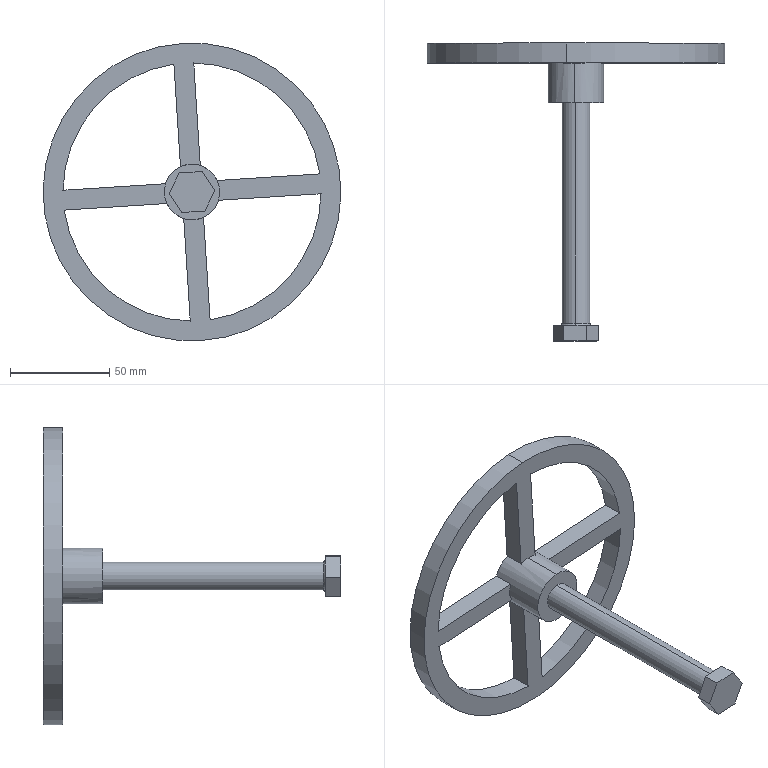Component | SolidWorks | adjuster roll-1 | 1 solid | 31 faces | box 150 x 150 x 150 mm | volume 102973 mm3 | plane 19 | cylinder 10 | torus 2 | commonest cylinder face diameters 130 x4 150 x2 28 x2 14 x2
STEP:
#1=COLOUR_RGB('',0.7922,0.8196,0.9333);
#2=FILL_AREA_STYLE_COLOUR('',#1);
#3=FILL_AREA_STYLE('',(#2));
#4=SURFACE_STYLE_FILL_AREA(#3);
#5=SURFACE_SIDE_STYLE('',(#4));
#6=SURFACE_STYLE_USAGE(.BOTH.,#5);
#7=PRESENTATION_STYLE_ASSIGNMENT((#6));
#8=CARTESIAN_POINT('',(-0.01998,5.433,1.102));
#9=VERTEX_POINT('',#8);
#10=CARTESIAN_POINT('',(0.01998,5.433,0.4731));
#11=VERTEX_POINT('',#10);
#12=CARTESIAN_POINT('',(0.,5.433,0.7874));
#13=DIRECTION('',(0.,-1.,0.));
#14=DIRECTION('',(0.06342,0.,-0.998));
#15=AXIS2_PLACEMENT_3D('',#12,#13,#14);
#16=CIRCLE('',#15,0.315);
#17=EDGE_CURVE('',#9,#11,#16,.T.);
#18=ORIENTED_EDGE('',*,*,#17,.F.);
#19=CARTESIAN_POINT('',(-0.01748,5.472,1.062));
#20=VERTEX_POINT('',#19);
#21=CARTESIAN_POINT('',(-0.01998,5.472,1.102));
#22=DIRECTION('',(0.998,0.,0.06342));
#23=DIRECTION('',(0.06342,0.,-0.998));
#24=AXIS2_PLACEMENT_3D('',#21,#22,#23);
#25=CIRCLE('',#24,0.03937);
#26=EDGE_CURVE('',#9,#20,#25,.T.);
#27=ORIENTED_EDGE('',*,*,#26,.T.);
#28=CARTESIAN_POINT('',(0.01748,5.472,0.5124));
#29=VERTEX_POINT('',#28);
#30=CARTESIAN_POINT('',(0.,5.472,0.7874));
#31=DIRECTION('',(0.,1.,0.));
#32=DIRECTION('',(0.06342,0.,-0.998));
#33=AXIS2_PLACEMENT_3D('',#30,#31,#32);
#34=CIRCLE('',#33,0.2756);
#35=EDGE_CURVE('',#29,#20,#34,.T.);
#36=ORIENTED_EDGE('',*,*,#35,.F.);
#37=CARTESIAN_POINT('',(0.01998,5.472,0.4731));
#38=DIRECTION('',(-0.998,0.,-0.06342));
#39=DIRECTION('',(-0.06342,0.,0.998));
#40=AXIS2_PLACEMENT_3D('',#37,#38,#39);
#41=CIRCLE('',#40,0.03937);
#42=EDGE_CURVE('',#11,#29,#41,.T.);
#43=ORIENTED_EDGE('',*,*,#42,.F.);
#44=EDGE_LOOP('',(#18,#27,#36,#43));
#45=FACE_OUTER_BOUND('',#44,.T.);
#46=CARTESIAN_POINT('',(0.,5.472,0.7874));
#47=DIRECTION('',(0.,-1.,0.));
#48=DIRECTION('',(0.06342,0.,-0.998));
#49=AXIS2_PLACEMENT_3D('',#46,#47,#48);
#50=TOROIDAL_SURFACE('',#49,0.315,0.03937);
#51=ADVANCED_FACE('',(#45),#50,.F.);
#52=CARTESIAN_POINT('',(-0.1873,11.024,3.734));
#53=VERTEX_POINT('',#52);
#54=CARTESIAN_POINT('',(0.1873,11.024,-2.159));
#55=VERTEX_POINT('',#54);
#56=CARTESIAN_POINT('',(0.,11.024,0.7874));
#57=DIRECTION('',(0.,1.,0.));
#58=DIRECTION('',(-0.06342,0.,0.998));
#59=AXIS2_PLACEMENT_3D('',#56,#57,#58);
#60=CIRCLE('',#59,2.953);
#61=EDGE_CURVE('',#53,#55,#60,.T.);
#62=ORIENTED_EDGE('',*,*,#61,.F.);
#63=CARTESIAN_POINT('',(-0.1873,10.63,3.734));
#64=VERTEX_POINT('',#63);
#65=CARTESIAN_POINT('',(-0.1873,11.024,3.734));
#66=DIRECTION('',(0.,-1.,0.));
#67=VECTOR('',#66,39.37);
#68=LINE('',#65,#67);
#69=EDGE_CURVE('',#53,#64,#68,.T.);
#70=ORIENTED_EDGE('',*,*,#69,.T.);
#71=CARTESIAN_POINT('',(0.1873,10.63,-2.159));
#72=VERTEX_POINT('',#71);
#73=CARTESIAN_POINT('',(0.,10.63,0.7874));
#74=DIRECTION('',(0.,1.,0.));
#75=DIRECTION('',(-0.06342,0.,0.998));
#76=AXIS2_PLACEMENT_3D('',#73,#74,#75);
#77=CIRCLE('',#76,2.953);
#78=EDGE_CURVE('',#64,#72,#77,.T.);
#79=ORIENTED_EDGE('',*,*,#78,.T.);
#80=CARTESIAN_POINT('',(0.1873,11.024,-2.159));
#81=DIRECTION('',(0.,-1.,0.));
#82=VECTOR('',#81,39.37);
#83=LINE('',#80,#82);
#84=EDGE_CURVE('',#55,#72,#83,.T.);
#85=ORIENTED_EDGE('',*,*,#84,.F.);
#86=EDGE_LOOP('',(#62,#70,#79,#85));
#87=FACE_OUTER_BOUND('',#86,.T.);
#88=CARTESIAN_POINT('',(0.,11.024,0.7874));
#89=DIRECTION('',(0.,-1.,0.));
#90=DIRECTION('',(0.06342,0.,-0.998));
#91=AXIS2_PLACEMENT_3D('',#88,#89,#90);
#92=CYLINDRICAL_SURFACE('',#91,2.953);
#93=ADVANCED_FACE('',(#87),#92,.T.);
#94=CARTESIAN_POINT('',(-0.03496,10.63,1.337));
#95=VERTEX_POINT('',#94);
#96=CARTESIAN_POINT('',(0.1638,10.63,1.314));
#97=VERTEX_POINT('',#96);
#98=CARTESIAN_POINT('',(0.,10.63,0.7874));
#99=DIRECTION('',(0.,1.,0.));
#100=DIRECTION('',(-0.06342,0.,0.998));
#101=AXIS2_PLACEMENT_3D('',#98,#99,#100);
#102=CIRCLE('',#101,0.5512);
#103=EDGE_CURVE('',#95,#97,#102,.T.);
#104=ORIENTED_EDGE('',*,*,#103,.F.);
#105=CARTESIAN_POINT('',(-0.03496,9.843,1.337));
#106=VERTEX_POINT('',#105);
#107=CARTESIAN_POINT('',(-0.03496,10.63,1.337));
#108=DIRECTION('',(0.,-1.,0.));
#109=VECTOR('',#108,39.37);
#110=LINE('',#107,#109);
#111=EDGE_CURVE('',#95,#106,#110,.T.);
#112=ORIENTED_EDGE('',*,*,#111,.T.);
#113=CARTESIAN_POINT('',(0.03496,9.843,0.2373));
#114=VERTEX_POINT('',#113);
#115=CARTESIAN_POINT('',(0.,9.843,0.7874));
#116=DIRECTION('',(0.,1.,0.));
#117=DIRECTION('',(-0.06342,0.,0.998));
#118=AXIS2_PLACEMENT_3D('',#115,#116,#117);
#119=CIRCLE('',#118,0.5512);
#120=EDGE_CURVE('',#106,#114,#119,.T.);
#121=ORIENTED_EDGE('',*,*,#120,.T.);
#122=CARTESIAN_POINT('',(0.03496,10.63,0.2373));
#123=VERTEX_POINT('',#122);
#124=CARTESIAN_POINT('',(0.03496,10.63,0.2373));
#125=DIRECTION('',(0.,-1.,0.));
#126=VECTOR('',#125,39.37);
#127=LINE('',#124,#126);
#128=EDGE_CURVE('',#123,#114,#127,.T.);
#129=ORIENTED_EDGE('',*,*,#128,.F.);
#130=CARTESIAN_POINT('',(0.2291,10.63,0.2861));
#131=VERTEX_POINT('',#130);
#132=CARTESIAN_POINT('',(0.,10.63,0.7874));
#133=DIRECTION('',(0.,1.,0.));
#134=DIRECTION('',(-0.06342,0.,0.998));
#135=AXIS2_PLACEMENT_3D('',#132,#133,#134);
#136=CIRCLE('',#135,0.5512);
#137=EDGE_CURVE('',#131,#123,#136,.T.);
#138=ORIENTED_EDGE('',*,*,#137,.F.);
#139=CARTESIAN_POINT('',(0.2291,11.024,0.2861));
#140=VERTEX_POINT('',#139);
#141=CARTESIAN_POINT('',(0.2291,11.024,0.2861));
#142=DIRECTION('',(0.,-1.,0.));
#143=VECTOR('',#142,39.37);
#144=LINE('',#141,#143);
#145=EDGE_CURVE('',#140,#131,#144,.T.);
#146=ORIENTED_EDGE('',*,*,#145,.F.);
#147=CARTESIAN_POINT('',(0.5263,11.024,0.6236));
#148=VERTEX_POINT('',#147);
#149=CARTESIAN_POINT('',(0.,11.024,0.7874));
#150=DIRECTION('',(0.,1.,0.));
#151=DIRECTION('',(-0.06342,0.,0.998));
#152=AXIS2_PLACEMENT_3D('',#149,#150,#151);
#153=CIRCLE('',#152,0.5512);
#154=EDGE_CURVE('',#148,#140,#153,.T.);
#155=ORIENTED_EDGE('',*,*,#154,.F.);
#156=CARTESIAN_POINT('',(0.5263,10.63,0.6236));
#157=VERTEX_POINT('',#156);
#158=CARTESIAN_POINT('',(0.5263,11.024,0.6236));
#159=DIRECTION('',(0.,-1.,0.));
#160=VECTOR('',#159,39.37);
#161=LINE('',#158,#160);
#162=EDGE_CURVE('',#148,#157,#161,.T.);
#163=ORIENTED_EDGE('',*,*,#162,.T.);
#164=CARTESIAN_POINT('',(0.5013,10.63,1.017));
#165=VERTEX_POINT('',#164);
#166=CARTESIAN_POINT('',(0.,10.63,0.7874));
#167=DIRECTION('',(0.,1.,0.));
#168=DIRECTION('',(-0.06342,0.,0.998));
#169=AXIS2_PLACEMENT_3D('',#166,#167,#168);
#170=CIRCLE('',#169,0.5512);
#171=EDGE_CURVE('',#165,#157,#170,.T.);
#172=ORIENTED_EDGE('',*,*,#171,.F.);
#173=CARTESIAN_POINT('',(0.5013,11.024,1.017));
#174=VERTEX_POINT('',#173);
#175=CARTESIAN_POINT('',(0.5013,11.024,1.017));
#176=DIRECTION('',(0.,-1.,0.));
#177=VECTOR('',#176,39.37);
#178=LINE('',#175,#177);
#179=EDGE_CURVE('',#174,#165,#178,.T.);
#180=ORIENTED_EDGE('',*,*,#179,.F.);
#181=CARTESIAN_POINT('',(0.1638,11.024,1.314));
#182=VERTEX_POINT('',#181);
#183=CARTESIAN_POINT('',(0.,11.024,0.7874));
#184=DIRECTION('',(0.,1.,0.));
#185=DIRECTION('',(-0.06342,0.,0.998));
#186=AXIS2_PLACEMENT_3D('',#183,#184,#185);
#187=CIRCLE('',#186,0.5512);
#188=EDGE_CURVE('',#182,#174,#187,.T.);
#189=ORIENTED_EDGE('',*,*,#188,.F.);
#190=CARTESIAN_POINT('',(0.1638,11.024,1.314));
#191=DIRECTION('',(0.,-1.,0.));
#192=VECTOR('',#191,39.37);
#193=LINE('',#190,#192);
#194=EDGE_CURVE('',#182,#97,#193,.T.);
#195=ORIENTED_EDGE('',*,*,#194,.T.);
#196=EDGE_LOOP('',(#104,#112,#121,#129,#138,#146,#155,#163,#172,#180,#189,#195));
#197=FACE_OUTER_BOUND('',#196,.T.);
#198=CARTESIAN_POINT('',(0.,10.63,0.7874));
#199=DIRECTION('',(0.,-1.,0.));
#200=DIRECTION('',(0.06342,0.,-0.998));
#201=AXIS2_PLACEMENT_3D('',#198,#199,#200);
#202=CYLINDRICAL_SURFACE('',#201,0.5512);
#203=ADVANCED_FACE('',(#197),#202,.T.);
#204=CARTESIAN_POINT('',(-0.01748,9.843,1.062));
#205=VERTEX_POINT('',#204);
#206=CARTESIAN_POINT('',(0.01748,9.843,0.5124));
#207=VERTEX_POINT('',#206);
#208=CARTESIAN_POINT('',(0.,9.843,0.7874));
#209=DIRECTION('',(0.,1.,0.));
#210=DIRECTION('',(-0.06342,0.,0.998));
#211=AXIS2_PLACEMENT_3D('',#208,#209,#210);
#212=CIRCLE('',#211,0.2756);
#213=EDGE_CURVE('',#205,#207,#212,.T.);
#214=ORIENTED_EDGE('',*,*,#213,.F.);
#215=CARTESIAN_POINT('',(-0.01748,9.843,1.062));
#216=DIRECTION('',(0.,-1.,0.));
#217=VECTOR('',#216,39.37);
#218=LINE('',#215,#217);
#219=EDGE_CURVE('',#205,#20,#218,.T.);
#220=ORIENTED_EDGE('',*,*,#219,.T.);
#221=CARTESIAN_POINT('',(0.,5.472,0.7874));
#222=DIRECTION('',(0.,1.,0.));
#223=DIRECTION('',(0.06342,0.,-0.998));
#224=AXIS2_PLACEMENT_3D('',#221,#222,#223);
#225=CIRCLE('',#224,0.2756);
#226=EDGE_CURVE('',#20,#29,#225,.T.);
#227=ORIENTED_EDGE('',*,*,#226,.T.);
#228=CARTESIAN_POINT('',(0.01748,9.843,0.5124));
#229=DIRECTION('',(0.,-1.,0.));
#230=VECTOR('',#229,39.37);
#231=LINE('',#228,#230);
#232=EDGE_CURVE('',#207,#29,#231,.T.);
#233=ORIENTED_EDGE('',*,*,#232,.F.);
#234=EDGE_LOOP('',(#214,#220,#227,#233));
#235=FACE_OUTER_BOUND('',#234,.T.);
#236=CARTESIAN_POINT('',(0.,9.843,0.7874));
#237=DIRECTION('',(0.,-1.,0.));
#238=DIRECTION('',(0.06342,0.,-0.998));
#239=AXIS2_PLACEMENT_3D('',#236,#237,#238);
#240=CYLINDRICAL_SURFACE('',#239,0.2756);
#241=ADVANCED_FACE('',(#235),#240,.T.);
#242=CARTESIAN_POINT('',(-0.1638,11.024,0.2611));
#243=VERTEX_POINT('',#242);
#244=CARTESIAN_POINT('',(-0.1638,10.63,0.2611));
#245=VERTEX_POINT('',#244);
#246=CARTESIAN_POINT('',(-0.1638,11.024,0.2611));
#247=DIRECTION('',(0.,-1.,0.));
#248=VECTOR('',#247,39.37);
#249=LINE('',#246,#248);
#250=EDGE_CURVE('',#243,#245,#249,.T.);
#251=ORIENTED_EDGE('',*,*,#250,.F.);
#252=CARTESIAN_POINT('',(-0.03463,11.024,-1.771));
#253=VERTEX_POINT('',#252);
#254=CARTESIAN_POINT('',(-0.1965,11.024,0.7749));
#255=DIRECTION('',(0.06342,0.,-0.998));
#256=VECTOR('',#255,39.37);
#257=LINE('',#254,#256);
#258=EDGE_CURVE('',#243,#253,#257,.T.);
#259=ORIENTED_EDGE('',*,*,#258,.T.);
#260=CARTESIAN_POINT('',(-0.03463,10.63,-1.771));
#261=VERTEX_POINT('',#260);
#262=CARTESIAN_POINT('',(-0.03463,7.3,-1.771));
#263=DIRECTION('',(0.,1.,0.));
#264=VECTOR('',#263,39.37);
#265=LINE('',#262,#264);
#266=EDGE_CURVE('',#261,#253,#265,.T.);
#267=ORIENTED_EDGE('',*,*,#266,.F.);
#268=CARTESIAN_POINT('',(-0.1965,10.63,0.7749));
#269=DIRECTION('',(-0.06342,0.,0.998));
#270=VECTOR('',#269,39.37);
#271=LINE('',#268,#270);
#272=EDGE_CURVE('',#261,#245,#271,.T.);
#273=ORIENTED_EDGE('',*,*,#272,.T.);
#274=EDGE_LOOP('',(#251,#259,#267,#273));
#275=FACE_OUTER_BOUND('',#274,.T.);
#276=CARTESIAN_POINT('',(-0.1965,7.3,0.7749));
#277=DIRECTION('',(0.998,0.,0.06342));
#278=DIRECTION('',(0.06342,0.,-0.998));
#279=AXIS2_PLACEMENT_3D('',#276,#277,#278);
#280=PLANE('',#279);
#281=ADVANCED_FACE('',(#275),#280,.F.);
#282=CARTESIAN_POINT('',(-0.5013,11.024,0.5583));
#283=VERTEX_POINT('',#282);
#284=CARTESIAN_POINT('',(-2.534,11.024,0.4291));
#285=VERTEX_POINT('',#284);
#286=CARTESIAN_POINT('',(0.01248,11.024,0.5909));
#287=DIRECTION('',(-0.998,0.,-0.06342));
#288=VECTOR('',#287,39.37);
#289=LINE('',#286,#288);
#290=EDGE_CURVE('',#283,#285,#289,.T.);
#291=ORIENTED_EDGE('',*,*,#290,.F.);
#292=CARTESIAN_POINT('',(-0.5013,10.63,0.5583));
#293=VERTEX_POINT('',#292);
#294=CARTESIAN_POINT('',(-0.5013,11.024,0.5583));
#295=DIRECTION('',(0.,-1.,0.));
#296=VECTOR('',#295,39.37);
#297=LINE('',#294,#296);
#298=EDGE_CURVE('',#283,#293,#297,.T.);
#299=ORIENTED_EDGE('',*,*,#298,.T.);
#300=CARTESIAN_POINT('',(-2.534,10.63,0.4291));
#301=VERTEX_POINT('',#300);
#302=CARTESIAN_POINT('',(0.01248,10.63,0.5909));
#303=DIRECTION('',(0.998,0.,0.06342));
#304=VECTOR('',#303,39.37);
#305=LINE('',#302,#304);
#306=EDGE_CURVE('',#301,#293,#305,.T.);
#307=ORIENTED_EDGE('',*,*,#306,.F.);
#308=CARTESIAN_POINT('',(-2.534,7.3,0.4291));
#309=DIRECTION('',(0.,1.,0.));
#310=VECTOR('',#309,39.37);
#311=LINE('',#308,#310);
#312=EDGE_CURVE('',#301,#285,#311,.T.);
#313=ORIENTED_EDGE('',*,*,#312,.T.);
#314=EDGE_LOOP('',(#291,#299,#307,#313));
#315=FACE_OUTER_BOUND('',#314,.T.);
#316=CARTESIAN_POINT('',(0.01248,7.3,0.5909));
#317=DIRECTION('',(0.06342,0.,-0.998));
#318=DIRECTION('',(-0.998,0.,-0.06342));
#319=AXIS2_PLACEMENT_3D('',#316,#317,#318);
#320=PLANE('',#319);
#321=ADVANCED_FACE('',(#315),#320,.T.);
#322=CARTESIAN_POINT('',(-0.5263,11.024,0.9512));
#323=VERTEX_POINT('',#322);
#324=CARTESIAN_POINT('',(-0.5263,10.63,0.9512));
#325=VERTEX_POINT('',#324);
#326=CARTESIAN_POINT('',(-0.5263,11.024,0.9512));
#327=DIRECTION('',(0.,-1.,0.));
#328=VECTOR('',#327,39.37);
#329=LINE('',#326,#328);
#330=EDGE_CURVE('',#323,#325,#329,.T.);
#331=ORIENTED_EDGE('',*,*,#330,.F.);
#332=CARTESIAN_POINT('',(-2.559,11.024,0.822));
#333=VERTEX_POINT('',#332);
#334=CARTESIAN_POINT('',(-0.01248,11.024,0.9839));
#335=DIRECTION('',(-0.998,0.,-0.06342));
#336=VECTOR('',#335,39.37);
#337=LINE('',#334,#336);
#338=EDGE_CURVE('',#323,#333,#337,.T.);
#339=ORIENTED_EDGE('',*,*,#338,.T.);
#340=CARTESIAN_POINT('',(-2.559,10.63,0.822));
#341=VERTEX_POINT('',#340);
#342=CARTESIAN_POINT('',(-2.559,7.3,0.822));
#343=DIRECTION('',(0.,1.,0.));
#344=VECTOR('',#343,39.37);
#345=LINE('',#342,#344);
#346=EDGE_CURVE('',#341,#333,#345,.T.);
#347=ORIENTED_EDGE('',*,*,#346,.F.);
#348=CARTESIAN_POINT('',(-0.01248,10.63,0.9839));
#349=DIRECTION('',(0.998,0.,0.06342));
#350=VECTOR('',#349,39.37);
#351=LINE('',#348,#350);
#352=EDGE_CURVE('',#341,#325,#351,.T.);
#353=ORIENTED_EDGE('',*,*,#352,.T.);
#354=EDGE_LOOP('',(#331,#339,#347,#353));
#355=FACE_OUTER_BOUND('',#354,.T.);
#356=CARTESIAN_POINT('',(-0.01248,7.3,0.9839));
#357=DIRECTION('',(0.06342,0.,-0.998));
#358=DIRECTION('',(-0.998,0.,-0.06342));
#359=AXIS2_PLACEMENT_3D('',#356,#357,#358);
#360=PLANE('',#359);
#361=ADVANCED_FACE('',(#355),#360,.F.);
#362=CARTESIAN_POINT('',(-0.2291,11.024,1.289));
#363=VERTEX_POINT('',#362);
#364=CARTESIAN_POINT('',(-0.3583,11.024,3.321));
#365=VERTEX_POINT('',#364);
#366=CARTESIAN_POINT('',(-0.1965,11.024,0.7749));
#367=DIRECTION('',(-0.06342,0.,0.998));
#368=VECTOR('',#367,39.37);
#369=LINE('',#366,#368);
#370=EDGE_CURVE('',#363,#365,#369,.T.);
#371=ORIENTED_EDGE('',*,*,#370,.F.);
#372=CARTESIAN_POINT('',(-0.2291,10.63,1.289));
#373=VERTEX_POINT('',#372);
#374=CARTESIAN_POINT('',(-0.2291,11.024,1.289));
#375=DIRECTION('',(0.,-1.,0.));
#376=VECTOR('',#375,39.37);
#377=LINE('',#374,#376);
#378=EDGE_CURVE('',#363,#373,#377,.T.);
#379=ORIENTED_EDGE('',*,*,#378,.T.);
#380=CARTESIAN_POINT('',(-0.3583,10.63,3.321));
#381=VERTEX_POINT('',#380);
#382=CARTESIAN_POINT('',(-0.1965,10.63,0.7749));
#383=DIRECTION('',(0.06342,0.,-0.998));
#384=VECTOR('',#383,39.37);
#385=LINE('',#382,#384);
#386=EDGE_CURVE('',#381,#373,#385,.T.);
#387=ORIENTED_EDGE('',*,*,#386,.F.);
#388=CARTESIAN_POINT('',(-0.3583,7.3,3.321));
#389=DIRECTION('',(0.,1.,0.));
#390=VECTOR('',#389,39.37);
#391=LINE('',#388,#390);
#392=EDGE_CURVE('',#381,#365,#391,.T.);
#393=ORIENTED_EDGE('',*,*,#392,.T.);
#394=EDGE_LOOP('',(#371,#379,#387,#393));
#395=FACE_OUTER_BOUND('',#394,.T.);
#396=CARTESIAN_POINT('',(-0.1965,7.3,0.7749));
#397=DIRECTION('',(-0.998,0.,-0.06342));
#398=DIRECTION('',(-0.06342,0.,0.998));
#399=AXIS2_PLACEMENT_3D('',#396,#397,#398);
#400=PLANE('',#399);
#401=ADVANCED_FACE('',(#395),#400,.T.);
#402=ORIENTED_EDGE('',*,*,#194,.F.);
#403=CARTESIAN_POINT('',(0.03463,11.024,3.346));
#404=VERTEX_POINT('',#403);
#405=CARTESIAN_POINT('',(0.1965,11.024,0.7999));
#406=DIRECTION('',(-0.06342,0.,0.998));
#407=VECTOR('',#406,39.37);
#408=LINE('',#405,#407);
#409=EDGE_CURVE('',#182,#404,#408,.T.);
#410=ORIENTED_EDGE('',*,*,#409,.T.);
#411=CARTESIAN_POINT('',(0.03463,10.63,3.346));
#412=VERTEX_POINT('',#411);
#413=CARTESIAN_POINT('',(0.03463,7.3,3.346));
#414=DIRECTION('',(0.,1.,0.));
#415=VECTOR('',#414,39.37);
#416=LINE('',#413,#415);
#417=EDGE_CURVE('',#412,#404,#416,.T.);
#418=ORIENTED_EDGE('',*,*,#417,.F.);
#419=CARTESIAN_POINT('',(0.1965,10.63,0.7999));
#420=DIRECTION('',(0.06342,0.,-0.998));
#421=VECTOR('',#420,39.37);
#422=LINE('',#419,#421);
#423=EDGE_CURVE('',#412,#97,#422,.T.);
#424=ORIENTED_EDGE('',*,*,#423,.T.);
#425=EDGE_LOOP('',(#402,#410,#418,#424));
#426=FACE_OUTER_BOUND('',#425,.T.);
#427=CARTESIAN_POINT('',(0.1965,7.3,0.7999));
#428=DIRECTION('',(-0.998,0.,-0.06342));
#429=DIRECTION('',(-0.06342,0.,0.998));
#430=AXIS2_PLACEMENT_3D('',#427,#428,#429);
#431=PLANE('',#430);
#432=ADVANCED_FACE('',(#426),#431,.F.);
#433=CARTESIAN_POINT('',(2.534,11.024,1.146));
#434=VERTEX_POINT('',#433);
#435=CARTESIAN_POINT('',(-0.01248,11.024,0.9839));
#436=DIRECTION('',(0.998,0.,0.06342));
#437=VECTOR('',#436,39.37);
#438=LINE('',#435,#437);
#439=EDGE_CURVE('',#174,#434,#438,.T.);
#440=ORIENTED_EDGE('',*,*,#439,.F.);
#441=ORIENTED_EDGE('',*,*,#179,.T.);
#442=CARTESIAN_POINT('',(2.534,10.63,1.146));
#443=VERTEX_POINT('',#442);
#444=CARTESIAN_POINT('',(-0.01248,10.63,0.9839));
#445=DIRECTION('',(-0.998,0.,-0.06342));
#446=VECTOR('',#445,39.37);
#447=LINE('',#444,#446);
#448=EDGE_CURVE('',#443,#165,#447,.T.);
#449=ORIENTED_EDGE('',*,*,#448,.F.);
#450=CARTESIAN_POINT('',(2.534,7.3,1.146));
#451=DIRECTION('',(0.,1.,0.));
#452=VECTOR('',#451,39.37);
#453=LINE('',#450,#452);
#454=EDGE_CURVE('',#443,#434,#453,.T.);
#455=ORIENTED_EDGE('',*,*,#454,.T.);
#456=EDGE_LOOP('',(#440,#441,#449,#455));
#457=FACE_OUTER_BOUND('',#456,.T.);
#458=CARTESIAN_POINT('',(-0.01248,7.3,0.9839));
#459=DIRECTION('',(-0.06342,0.,0.998));
#460=DIRECTION('',(0.998,0.,0.06342));
#461=AXIS2_PLACEMENT_3D('',#458,#459,#460);
#462=PLANE('',#461);
#463=ADVANCED_FACE('',(#457),#462,.T.);
#464=ORIENTED_EDGE('',*,*,#162,.F.);
#465=CARTESIAN_POINT('',(2.559,11.024,0.7528));
#466=VERTEX_POINT('',#465);
#467=CARTESIAN_POINT('',(0.01248,11.024,0.5909));
#468=DIRECTION('',(0.998,0.,0.06342));
#469=VECTOR('',#468,39.37);
#470=LINE('',#467,#469);
#471=EDGE_CURVE('',#148,#466,#470,.T.);
#472=ORIENTED_EDGE('',*,*,#471,.T.);
#473=CARTESIAN_POINT('',(2.559,10.63,0.7528));
#474=VERTEX_POINT('',#473);
#475=CARTESIAN_POINT('',(2.559,7.3,0.7528));
#476=DIRECTION('',(0.,1.,0.));
#477=VECTOR('',#476,39.37);
#478=LINE('',#475,#477);
#479=EDGE_CURVE('',#474,#466,#478,.T.);
#480=ORIENTED_EDGE('',*,*,#479,.F.);
#481=CARTESIAN_POINT('',(0.01248,10.63,0.5909));
#482=DIRECTION('',(-0.998,0.,-0.06342));
#483=VECTOR('',#482,39.37);
#484=LINE('',#481,#483);
#485=EDGE_CURVE('',#474,#157,#484,.T.);
#486=ORIENTED_EDGE('',*,*,#485,.T.);
#487=EDGE_LOOP('',(#464,#472,#480,#486));
#488=FACE_OUTER_BOUND('',#487,.T.);
#489=CARTESIAN_POINT('',(0.01248,7.3,0.5909));
#490=DIRECTION('',(-0.06342,0.,0.998));
#491=DIRECTION('',(0.998,0.,0.06342));
#492=AXIS2_PLACEMENT_3D('',#489,#490,#491);
#493=PLANE('',#492);
#494=ADVANCED_FACE('',(#488),#493,.F.);
#495=CARTESIAN_POINT('',(0.3583,11.024,-1.746));
#496=VERTEX_POINT('',#495);
#497=CARTESIAN_POINT('',(0.1965,11.024,0.7999));
#498=DIRECTION('',(0.06342,0.,-0.998));
#499=VECTOR('',#498,39.37);
#500=LINE('',#497,#499);
#501=EDGE_CURVE('',#140,#496,#500,.T.);
#502=ORIENTED_EDGE('',*,*,#501,.F.);
#503=ORIENTED_EDGE('',*,*,#145,.T.);
#504=CARTESIAN_POINT('',(0.3583,10.63,-1.746));
#505=VERTEX_POINT('',#504);
#506=CARTESIAN_POINT('',(0.1965,10.63,0.7999));
#507=DIRECTION('',(-0.06342,0.,0.998));
#508=VECTOR('',#507,39.37);
#509=LINE('',#506,#508);
#510=EDGE_CURVE('',#505,#131,#509,.T.);
#511=ORIENTED_EDGE('',*,*,#510,.F.);
#512=CARTESIAN_POINT('',(0.3583,7.3,-1.746));
#513=DIRECTION('',(0.,1.,0.));
#514=VECTOR('',#513,39.37);
#515=LINE('',#512,#514);
#516=EDGE_CURVE('',#505,#496,#515,.T.);
#517=ORIENTED_EDGE('',*,*,#516,.T.);
#518=EDGE_LOOP('',(#502,#503,#511,#517));
#519=FACE_OUTER_BOUND('',#518,.T.);
#520=CARTESIAN_POINT('',(0.1965,7.3,0.7999));
#521=DIRECTION('',(0.998,0.,0.06342));
#522=DIRECTION('',(0.06342,0.,-0.998));
#523=AXIS2_PLACEMENT_3D('',#520,#521,#522);
#524=PLANE('',#523);
#525=ADVANCED_FACE('',(#519),#524,.T.);
#526=ORIENTED_EDGE('',*,*,#219,.F.);
#527=CARTESIAN_POINT('',(0.,9.843,0.7874));
#528=DIRECTION('',(0.,1.,0.));
#529=DIRECTION('',(-0.06342,0.,0.998));
#530=AXIS2_PLACEMENT_3D('',#527,#528,#529);
#531=CIRCLE('',#530,0.2756);
#532=EDGE_CURVE('',#207,#205,#531,.T.);
#533=ORIENTED_EDGE('',*,*,#532,.F.);
#534=ORIENTED_EDGE('',*,*,#232,.T.);
#535=ORIENTED_EDGE('',*,*,#35,.T.);
#536=EDGE_LOOP('',(#526,#533,#534,#535));
#537=FACE_OUTER_BOUND('',#536,.T.);
#538=CARTESIAN_POINT('',(0.,9.843,0.7874));
#539=DIRECTION('',(0.,-1.,0.));
#540=DIRECTION('',(0.06342,0.,-0.998));
#541=AXIS2_PLACEMENT_3D('',#538,#539,#540);
#542=CYLINDRICAL_SURFACE('',#541,0.2756);
#543=ADVANCED_FACE('',(#537),#542,.T.);
#544=ORIENTED_EDGE('',*,*,#111,.F.);
#545=CARTESIAN_POINT('',(0.,10.63,0.7874));
#546=DIRECTION('',(0.,1.,0.));
#547=DIRECTION('',(-0.06342,0.,0.998));
#548=AXIS2_PLACEMENT_3D('',#545,#546,#547);
#549=CIRCLE('',#548,0.5512);
#550=EDGE_CURVE('',#373,#95,#549,.T.);
#551=ORIENTED_EDGE('',*,*,#550,.F.);
#552=ORIENTED_EDGE('',*,*,#378,.F.);
#553=CARTESIAN_POINT('',(0.,11.024,0.7874));
#554=DIRECTION('',(0.,1.,0.));
#555=DIRECTION('',(-0.06342,0.,0.998));
#556=AXIS2_PLACEMENT_3D('',#553,#554,#555);
#557=CIRCLE('',#556,0.5512);
#558=EDGE_CURVE('',#323,#363,#557,.T.);
#559=ORIENTED_EDGE('',*,*,#558,.F.);
#560=ORIENTED_EDGE('',*,*,#330,.T.);
#561=CARTESIAN_POINT('',(0.,10.63,0.7874));
#562=DIRECTION('',(0.,1.,0.));
#563=DIRECTION('',(-0.06342,0.,0.998));
#564=AXIS2_PLACEMENT_3D('',#561,#562,#563);
#565=CIRCLE('',#564,0.5512);
#566=EDGE_CURVE('',#293,#325,#565,.T.);
#567=ORIENTED_EDGE('',*,*,#566,.F.);
#568=ORIENTED_EDGE('',*,*,#298,.F.);
#569=CARTESIAN_POINT('',(0.,11.024,0.7874));
#570=DIRECTION('',(0.,1.,0.));
#571=DIRECTION('',(-0.06342,0.,0.998));
#572=AXIS2_PLACEMENT_3D('',#569,#570,#571);
#573=CIRCLE('',#572,0.5512);
#574=EDGE_CURVE('',#243,#283,#573,.T.);
#575=ORIENTED_EDGE('',*,*,#574,.F.);
#576=ORIENTED_EDGE('',*,*,#250,.T.);
#577=CARTESIAN_POINT('',(0.,10.63,0.7874));
#578=DIRECTION('',(0.,1.,0.));
#579=DIRECTION('',(-0.06342,0.,0.998));
#580=AXIS2_PLACEMENT_3D('',#577,#578,#579);
#581=CIRCLE('',#580,0.5512);
#582=EDGE_CURVE('',#123,#245,#581,.T.);
#583=ORIENTED_EDGE('',*,*,#582,.F.);
#584=ORIENTED_EDGE('',*,*,#128,.T.);
#585=CARTESIAN_POINT('',(0.,9.843,0.7874));
#586=DIRECTION('',(0.,1.,0.));
#587=DIRECTION('',(-0.06342,0.,0.998));
#588=AXIS2_PLACEMENT_3D('',#585,#586,#587);
#589=CIRCLE('',#588,0.5512);
#590=EDGE_CURVE('',#114,#106,#589,.T.);
#591=ORIENTED_EDGE('',*,*,#590,.T.);
#592=EDGE_LOOP('',(#544,#551,#552,#559,#560,#567,#568,#575,#576,#583,#584,#591));
#593=FACE_OUTER_BOUND('',#592,.T.);
#594=CARTESIAN_POINT('',(0.,10.63,0.7874));
#595=DIRECTION('',(0.,-1.,0.));
#596=DIRECTION('',(0.06342,0.,-0.998));
#597=AXIS2_PLACEMENT_3D('',#594,#595,#596);
#598=CYLINDRICAL_SURFACE('',#597,0.5512);
#599=ADVANCED_FACE('',(#593),#598,.T.);
#600=ORIENTED_EDGE('',*,*,#532,.T.);
#601=ORIENTED_EDGE('',*,*,#213,.T.);
#602=EDGE_LOOP('',(#600,#601));
#603=FACE_BOUND('',#602,.T.);
#604=ORIENTED_EDGE('',*,*,#590,.F.);
#605=ORIENTED_EDGE('',*,*,#120,.F.);
#606=EDGE_LOOP('',(#604,#605));
#607=FACE_OUTER_BOUND('',#606,.T.);
#608=CARTESIAN_POINT('',(0.,9.843,0.7874));
#609=DIRECTION('',(0.,1.,0.));
#610=DIRECTION('',(-0.06342,0.,0.998));
#611=AXIS2_PLACEMENT_3D('',#608,#609,#610);
#612=PLANE('',#611);
#613=ADVANCED_FACE('',(#603,#607),#612,.F.);
#614=ORIENTED_EDGE('',*,*,#69,.F.);
#615=CARTESIAN_POINT('',(0.,11.024,0.7874));
#616=DIRECTION('',(0.,1.,0.));
#617=DIRECTION('',(-0.06342,0.,0.998));
#618=AXIS2_PLACEMENT_3D('',#615,#616,#617);
#619=CIRCLE('',#618,2.953);
#620=EDGE_CURVE('',#55,#53,#619,.T.);
#621=ORIENTED_EDGE('',*,*,#620,.F.);
#622=ORIENTED_EDGE('',*,*,#84,.T.);
#623=CARTESIAN_POINT('',(0.,10.63,0.7874));
#624=DIRECTION('',(0.,1.,0.));
#625=DIRECTION('',(-0.06342,0.,0.998));
#626=AXIS2_PLACEMENT_3D('',#623,#624,#625);
#627=CIRCLE('',#626,2.953);
#628=EDGE_CURVE('',#72,#64,#627,.T.);
#629=ORIENTED_EDGE('',*,*,#628,.T.);
#630=EDGE_LOOP('',(#614,#621,#622,#629));
#631=FACE_OUTER_BOUND('',#630,.T.);
#632=CARTESIAN_POINT('',(0.,11.024,0.7874));
#633=DIRECTION('',(0.,-1.,0.));
#634=DIRECTION('',(0.06342,0.,-0.998));
#635=AXIS2_PLACEMENT_3D('',#632,#633,#634);
#636=CYLINDRICAL_SURFACE('',#635,2.953);
#637=ADVANCED_FACE('',(#631),#636,.T.);
#638=ORIENTED_EDGE('',*,*,#258,.F.);
#639=ORIENTED_EDGE('',*,*,#574,.T.);
#640=ORIENTED_EDGE('',*,*,#290,.T.);
#641=CARTESIAN_POINT('',(0.,11.024,0.7874));
#642=DIRECTION('',(0.,1.,0.));
#643=DIRECTION('',(-0.06342,0.,0.998));
#644=AXIS2_PLACEMENT_3D('',#641,#642,#643);
#645=CIRCLE('',#644,2.559);
#646=EDGE_CURVE('',#253,#285,#645,.T.);
#647=ORIENTED_EDGE('',*,*,#646,.F.);
#648=EDGE_LOOP('',(#638,#639,#640,#647));
#649=FACE_BOUND('',#648,.T.);
#650=ORIENTED_EDGE('',*,*,#338,.F.);
#651=ORIENTED_EDGE('',*,*,#558,.T.);
#652=ORIENTED_EDGE('',*,*,#370,.T.);
#653=CARTESIAN_POINT('',(0.,11.024,0.7874));
#654=DIRECTION('',(0.,1.,0.));
#655=DIRECTION('',(-0.06342,0.,0.998));
#656=AXIS2_PLACEMENT_3D('',#653,#654,#655);
#657=CIRCLE('',#656,2.559);
#658=EDGE_CURVE('',#333,#365,#657,.T.);
#659=ORIENTED_EDGE('',*,*,#658,.F.);
#660=EDGE_LOOP('',(#650,#651,#652,#659));
#661=FACE_BOUND('',#660,.T.);
#662=ORIENTED_EDGE('',*,*,#409,.F.);
#663=ORIENTED_EDGE('',*,*,#188,.T.);
#664=ORIENTED_EDGE('',*,*,#439,.T.);
#665=CARTESIAN_POINT('',(0.,11.024,0.7874));
#666=DIRECTION('',(0.,1.,0.));
#667=DIRECTION('',(-0.06342,0.,0.998));
#668=AXIS2_PLACEMENT_3D('',#665,#666,#667);
#669=CIRCLE('',#668,2.559);
#670=EDGE_CURVE('',#404,#434,#669,.T.);
#671=ORIENTED_EDGE('',*,*,#670,.F.);
#672=EDGE_LOOP('',(#662,#663,#664,#671));
#673=FACE_BOUND('',#672,.T.);
#674=ORIENTED_EDGE('',*,*,#471,.F.);
#675=ORIENTED_EDGE('',*,*,#154,.T.);
#676=ORIENTED_EDGE('',*,*,#501,.T.);
#677=CARTESIAN_POINT('',(0.,11.024,0.7874));
#678=DIRECTION('',(0.,1.,0.));
#679=DIRECTION('',(-0.06342,0.,0.998));
#680=AXIS2_PLACEMENT_3D('',#677,#678,#679);
#681=CIRCLE('',#680,2.559);
#682=EDGE_CURVE('',#466,#496,#681,.T.);
#683=ORIENTED_EDGE('',*,*,#682,.F.);
#684=EDGE_LOOP('',(#674,#675,#676,#683));
#685=FACE_BOUND('',#684,.T.);
#686=ORIENTED_EDGE('',*,*,#620,.T.);
#687=ORIENTED_EDGE('',*,*,#61,.T.);
#688=EDGE_LOOP('',(#686,#687));
#689=FACE_OUTER_BOUND('',#688,.T.);
#690=CARTESIAN_POINT('',(0.,11.024,0.7874));
#691=DIRECTION('',(0.,1.,0.));
#692=DIRECTION('',(-0.06342,0.,0.998));
#693=AXIS2_PLACEMENT_3D('',#690,#691,#692);
#694=PLANE('',#693);
#695=ADVANCED_FACE('',(#649,#661,#673,#685,#689),#694,.T.);
#696=ORIENTED_EDGE('',*,*,#566,.T.);
#697=ORIENTED_EDGE('',*,*,#352,.F.);
#698=CARTESIAN_POINT('',(0.,10.63,0.7874));
#699=DIRECTION('',(0.,-1.,0.));
#700=DIRECTION('',(-0.06342,0.,0.998));
#701=AXIS2_PLACEMENT_3D('',#698,#699,#700);
#702=CIRCLE('',#701,2.559);
#703=EDGE_CURVE('',#381,#341,#702,.T.);
#704=ORIENTED_EDGE('',*,*,#703,.F.);
#705=ORIENTED_EDGE('',*,*,#386,.T.);
#706=ORIENTED_EDGE('',*,*,#550,.T.);
#707=ORIENTED_EDGE('',*,*,#103,.T.);
#708=ORIENTED_EDGE('',*,*,#423,.F.);
#709=CARTESIAN_POINT('',(0.,10.63,0.7874));
#710=DIRECTION('',(0.,-1.,0.));
#711=DIRECTION('',(-0.06342,0.,0.998));
#712=AXIS2_PLACEMENT_3D('',#709,#710,#711);
#713=CIRCLE('',#712,2.559);
#714=EDGE_CURVE('',#443,#412,#713,.T.);
#715=ORIENTED_EDGE('',*,*,#714,.F.);
#716=ORIENTED_EDGE('',*,*,#448,.T.);
#717=ORIENTED_EDGE('',*,*,#171,.T.);
#718=ORIENTED_EDGE('',*,*,#485,.F.);
#719=CARTESIAN_POINT('',(0.,10.63,0.7874));
#720=DIRECTION('',(0.,-1.,0.));
#721=DIRECTION('',(-0.06342,0.,0.998));
#722=AXIS2_PLACEMENT_3D('',#719,#720,#721);
#723=CIRCLE('',#722,2.559);
#724=EDGE_CURVE('',#505,#474,#723,.T.);
#725=ORIENTED_EDGE('',*,*,#724,.F.);
#726=ORIENTED_EDGE('',*,*,#510,.T.);
#727=ORIENTED_EDGE('',*,*,#137,.T.);
#728=ORIENTED_EDGE('',*,*,#582,.T.);
#729=ORIENTED_EDGE('',*,*,#272,.F.);
#730=CARTESIAN_POINT('',(0.,10.63,0.7874));
#731=DIRECTION('',(0.,-1.,0.));
#732=DIRECTION('',(-0.06342,0.,0.998));
#733=AXIS2_PLACEMENT_3D('',#730,#731,#732);
#734=CIRCLE('',#733,2.559);
#735=EDGE_CURVE('',#301,#261,#734,.T.);
#736=ORIENTED_EDGE('',*,*,#735,.F.);
#737=ORIENTED_EDGE('',*,*,#306,.T.);
#738=EDGE_LOOP('',(#696,#697,#704,#705,#706,#707,#708,#715,#716,#717,#718,#725,#726,#727,#728,#729,#736,#737));
#739=FACE_BOUND('',#738,.T.);
#740=ORIENTED_EDGE('',*,*,#628,.F.);
#741=ORIENTED_EDGE('',*,*,#78,.F.);
#742=EDGE_LOOP('',(#740,#741));
#743=FACE_OUTER_BOUND('',#742,.T.);
#744=CARTESIAN_POINT('',(0.,10.63,0.7874));
#745=DIRECTION('',(0.,1.,0.));
#746=DIRECTION('',(-0.06342,0.,0.998));
#747=AXIS2_PLACEMENT_3D('',#744,#745,#746);
#748=PLANE('',#747);
#749=ADVANCED_FACE('',(#739,#743),#748,.F.);
#750=ORIENTED_EDGE('',*,*,#714,.T.);
#751=ORIENTED_EDGE('',*,*,#417,.T.);
#752=ORIENTED_EDGE('',*,*,#670,.T.);
#753=ORIENTED_EDGE('',*,*,#454,.F.);
#754=EDGE_LOOP('',(#750,#751,#752,#753));
#755=FACE_OUTER_BOUND('',#754,.T.);
#756=CARTESIAN_POINT('',(0.,7.3,0.7874));
#757=DIRECTION('',(0.,1.,0.));
#758=DIRECTION('',(-0.06342,0.,0.998));
#759=AXIS2_PLACEMENT_3D('',#756,#757,#758);
#760=CYLINDRICAL_SURFACE('',#759,2.559);
#761=ADVANCED_FACE('',(#755),#760,.F.);
#762=ORIENTED_EDGE('',*,*,#724,.T.);
#763=ORIENTED_EDGE('',*,*,#479,.T.);
#764=ORIENTED_EDGE('',*,*,#682,.T.);
#765=ORIENTED_EDGE('',*,*,#516,.F.);
#766=EDGE_LOOP('',(#762,#763,#764,#765));
#767=FACE_OUTER_BOUND('',#766,.T.);
#768=CARTESIAN_POINT('',(0.,7.3,0.7874));
#769=DIRECTION('',(0.,1.,0.));
#770=DIRECTION('',(-0.06342,0.,0.998));
#771=AXIS2_PLACEMENT_3D('',#768,#769,#770);
#772=CYLINDRICAL_SURFACE('',#771,2.559);
#773=ADVANCED_FACE('',(#767),#772,.F.);
#774=ORIENTED_EDGE('',*,*,#735,.T.);
#775=ORIENTED_EDGE('',*,*,#266,.T.);
#776=ORIENTED_EDGE('',*,*,#646,.T.);
#777=ORIENTED_EDGE('',*,*,#312,.F.);
#778=EDGE_LOOP('',(#774,#775,#776,#777));
#779=FACE_OUTER_BOUND('',#778,.T.);
#780=CARTESIAN_POINT('',(0.,7.3,0.7874));
#781=DIRECTION('',(0.,1.,0.));
#782=DIRECTION('',(-0.06342,0.,0.998));
#783=AXIS2_PLACEMENT_3D('',#780,#781,#782);
#784=CYLINDRICAL_SURFACE('',#783,2.559);
#785=ADVANCED_FACE('',(#779),#784,.F.);
#786=ORIENTED_EDGE('',*,*,#703,.T.);
#787=ORIENTED_EDGE('',*,*,#346,.T.);
#788=ORIENTED_EDGE('',*,*,#658,.T.);
#789=ORIENTED_EDGE('',*,*,#392,.F.);
#790=EDGE_LOOP('',(#786,#787,#788,#789));
#791=FACE_OUTER_BOUND('',#790,.T.);
#792=CARTESIAN_POINT('',(0.,7.3,0.7874));
#793=DIRECTION('',(0.,1.,0.));
#794=DIRECTION('',(-0.06342,0.,0.998));
#795=AXIS2_PLACEMENT_3D('',#792,#793,#794);
#796=CYLINDRICAL_SURFACE('',#795,2.559);
#797=ADVANCED_FACE('',(#791),#796,.F.);
#798=CARTESIAN_POINT('',(0.4539,5.433,0.8127));
#799=VERTEX_POINT('',#798);
#800=CARTESIAN_POINT('',(0.205,5.433,1.193));
#801=VERTEX_POINT('',#800);
#802=CARTESIAN_POINT('',(0.4539,5.433,0.8127));
#803=DIRECTION('',(-0.5475,0.,0.8368));
#804=VECTOR('',#803,39.37);
#805=LINE('',#802,#804);
#806=EDGE_CURVE('',#799,#801,#805,.T.);
#807=ORIENTED_EDGE('',*,*,#806,.T.);
#808=CARTESIAN_POINT('',(0.205,5.118,1.193));
#809=VERTEX_POINT('',#808);
#810=CARTESIAN_POINT('',(0.205,5.118,1.193));
#811=DIRECTION('',(0.,1.,0.));
#812=VECTOR('',#811,39.37);
#813=LINE('',#810,#812);
#814=EDGE_CURVE('',#809,#801,#813,.T.);
#815=ORIENTED_EDGE('',*,*,#814,.F.);
#816=CARTESIAN_POINT('',(0.4539,5.118,0.8127));
#817=VERTEX_POINT('',#816);
#818=CARTESIAN_POINT('',(0.4539,5.118,0.8127));
#819=DIRECTION('',(-0.5475,0.,0.8368));
#820=VECTOR('',#819,39.37);
#821=LINE('',#818,#820);
#822=EDGE_CURVE('',#817,#809,#821,.T.);
#823=ORIENTED_EDGE('',*,*,#822,.F.);
#824=CARTESIAN_POINT('',(0.4539,5.118,0.8127));
#825=DIRECTION('',(0.,1.,0.));
#826=VECTOR('',#825,39.37);
#827=LINE('',#824,#826);
#828=EDGE_CURVE('',#817,#799,#827,.T.);
#829=ORIENTED_EDGE('',*,*,#828,.T.);
#830=EDGE_LOOP('',(#807,#815,#823,#829));
#831=FACE_OUTER_BOUND('',#830,.T.);
#832=CARTESIAN_POINT('',(0.4539,5.118,0.8127));
#833=DIRECTION('',(-0.8368,0.,-0.5475));
#834=DIRECTION('',(-0.5475,0.,0.8368));
#835=AXIS2_PLACEMENT_3D('',#832,#833,#834);
#836=PLANE('',#835);
#837=ADVANCED_FACE('',(#831),#836,.F.);
#838=CARTESIAN_POINT('',(-0.2489,5.433,1.168));
#839=VERTEX_POINT('',#838);
#840=CARTESIAN_POINT('',(0.205,5.433,1.193));
#841=DIRECTION('',(-0.9984,0.,-0.05572));
#842=VECTOR('',#841,39.37);
#843=LINE('',#840,#842);
#844=EDGE_CURVE('',#801,#839,#843,.T.);
#845=ORIENTED_EDGE('',*,*,#844,.T.);
#846=CARTESIAN_POINT('',(-0.2489,5.118,1.168));
#847=VERTEX_POINT('',#846);
#848=CARTESIAN_POINT('',(-0.2489,5.118,1.168));
#849=DIRECTION('',(0.,1.,0.));
#850=VECTOR('',#849,39.37);
#851=LINE('',#848,#850);
#852=EDGE_CURVE('',#847,#839,#851,.T.);
#853=ORIENTED_EDGE('',*,*,#852,.F.);
#854=CARTESIAN_POINT('',(0.205,5.118,1.193));
#855=DIRECTION('',(-0.9984,0.,-0.05572));
#856=VECTOR('',#855,39.37);
#857=LINE('',#854,#856);
#858=EDGE_CURVE('',#809,#847,#857,.T.);
#859=ORIENTED_EDGE('',*,*,#858,.F.);
#860=ORIENTED_EDGE('',*,*,#814,.T.);
#861=EDGE_LOOP('',(#845,#853,#859,#860));
#862=FACE_OUTER_BOUND('',#861,.T.);
#863=CARTESIAN_POINT('',(0.205,5.118,1.193));
#864=DIRECTION('',(0.05572,0.,-0.9984));
#865=DIRECTION('',(-0.9984,0.,-0.05572));
#866=AXIS2_PLACEMENT_3D('',#863,#864,#865);
#867=PLANE('',#866);
#868=ADVANCED_FACE('',(#862),#867,.F.);
#869=CARTESIAN_POINT('',(-0.4539,5.433,0.7621));
#870=VERTEX_POINT('',#869);
#871=CARTESIAN_POINT('',(-0.2489,5.433,1.168));
#872=DIRECTION('',(-0.451,0.,-0.8925));
#873=VECTOR('',#872,39.37);
#874=LINE('',#871,#873);
#875=EDGE_CURVE('',#839,#870,#874,.T.);
#876=ORIENTED_EDGE('',*,*,#875,.T.);
#877=CARTESIAN_POINT('',(-0.4539,5.118,0.7621));
#878=VERTEX_POINT('',#877);
#879=CARTESIAN_POINT('',(-0.4539,5.118,0.7621));
#880=DIRECTION('',(0.,1.,0.));
#881=VECTOR('',#880,39.37);
#882=LINE('',#879,#881);
#883=EDGE_CURVE('',#878,#870,#882,.T.);
#884=ORIENTED_EDGE('',*,*,#883,.F.);
#885=CARTESIAN_POINT('',(-0.2489,5.118,1.168));
#886=DIRECTION('',(-0.451,0.,-0.8925));
#887=VECTOR('',#886,39.37);
#888=LINE('',#885,#887);
#889=EDGE_CURVE('',#847,#878,#888,.T.);
#890=ORIENTED_EDGE('',*,*,#889,.F.);
#891=ORIENTED_EDGE('',*,*,#852,.T.);
#892=EDGE_LOOP('',(#876,#884,#890,#891));
#893=FACE_OUTER_BOUND('',#892,.T.);
#894=CARTESIAN_POINT('',(-0.2489,5.118,1.168));
#895=DIRECTION('',(0.8925,0.,-0.451));
#896=DIRECTION('',(-0.451,0.,-0.8925));
#897=AXIS2_PLACEMENT_3D('',#894,#895,#896);
#898=PLANE('',#897);
#899=ADVANCED_FACE('',(#893),#898,.F.);
#900=CARTESIAN_POINT('',(-0.205,5.433,0.3816));
#901=VERTEX_POINT('',#900);
#902=CARTESIAN_POINT('',(-0.4539,5.433,0.7621));
#903=DIRECTION('',(0.5475,0.,-0.8368));
#904=VECTOR('',#903,39.37);
#905=LINE('',#902,#904);
#906=EDGE_CURVE('',#870,#901,#905,.T.);
#907=ORIENTED_EDGE('',*,*,#906,.T.);
#908=CARTESIAN_POINT('',(-0.205,5.118,0.3816));
#909=VERTEX_POINT('',#908);
#910=CARTESIAN_POINT('',(-0.205,5.118,0.3816));
#911=DIRECTION('',(0.,1.,0.));
#912=VECTOR('',#911,39.37);
#913=LINE('',#910,#912);
#914=EDGE_CURVE('',#909,#901,#913,.T.);
#915=ORIENTED_EDGE('',*,*,#914,.F.);
#916=CARTESIAN_POINT('',(-0.4539,5.118,0.7621));
#917=DIRECTION('',(0.5475,0.,-0.8368));
#918=VECTOR('',#917,39.37);
#919=LINE('',#916,#918);
#920=EDGE_CURVE('',#878,#909,#919,.T.);
#921=ORIENTED_EDGE('',*,*,#920,.F.);
#922=ORIENTED_EDGE('',*,*,#883,.T.);
#923=EDGE_LOOP('',(#907,#915,#921,#922));
#924=FACE_OUTER_BOUND('',#923,.T.);
#925=CARTESIAN_POINT('',(-0.4539,5.118,0.7621));
#926=DIRECTION('',(0.8368,0.,0.5475));
#927=DIRECTION('',(0.5475,0.,-0.8368));
#928=AXIS2_PLACEMENT_3D('',#925,#926,#927);
#929=PLANE('',#928);
#930=ADVANCED_FACE('',(#924),#929,.F.);
#931=CARTESIAN_POINT('',(0.2489,5.433,0.407));
#932=VERTEX_POINT('',#931);
#933=CARTESIAN_POINT('',(-0.205,5.433,0.3816));
#934=DIRECTION('',(0.9984,0.,0.05572));
#935=VECTOR('',#934,39.37);
#936=LINE('',#933,#935);
#937=EDGE_CURVE('',#901,#932,#936,.T.);
#938=ORIENTED_EDGE('',*,*,#937,.T.);
#939=CARTESIAN_POINT('',(0.2489,5.118,0.407));
#940=VERTEX_POINT('',#939);
#941=CARTESIAN_POINT('',(0.2489,5.118,0.407));
#942=DIRECTION('',(0.,1.,0.));
#943=VECTOR('',#942,39.37);
#944=LINE('',#941,#943);
#945=EDGE_CURVE('',#940,#932,#944,.T.);
#946=ORIENTED_EDGE('',*,*,#945,.F.);
#947=CARTESIAN_POINT('',(-0.205,5.118,0.3816));
#948=DIRECTION('',(0.9984,0.,0.05572));
#949=VECTOR('',#948,39.37);
#950=LINE('',#947,#949);
#951=EDGE_CURVE('',#909,#940,#950,.T.);
#952=ORIENTED_EDGE('',*,*,#951,.F.);
#953=ORIENTED_EDGE('',*,*,#914,.T.);
#954=EDGE_LOOP('',(#938,#946,#952,#953));
#955=FACE_OUTER_BOUND('',#954,.T.);
#956=CARTESIAN_POINT('',(-0.205,5.118,0.3816));
#957=DIRECTION('',(-0.05572,0.,0.9984));
#958=DIRECTION('',(0.9984,0.,0.05572));
#959=AXIS2_PLACEMENT_3D('',#956,#957,#958);
#960=PLANE('',#959);
#961=ADVANCED_FACE('',(#955),#960,.F.);
#962=CARTESIAN_POINT('',(0.2489,5.433,0.407));
#963=DIRECTION('',(0.451,0.,0.8925));
#964=VECTOR('',#963,39.37);
#965=LINE('',#962,#964);
#966=EDGE_CURVE('',#932,#799,#965,.T.);
#967=ORIENTED_EDGE('',*,*,#966,.T.);
#968=ORIENTED_EDGE('',*,*,#828,.F.);
#969=CARTESIAN_POINT('',(0.2489,5.118,0.407));
#970=DIRECTION('',(0.451,0.,0.8925));
#971=VECTOR('',#970,39.37);
#972=LINE('',#969,#971);
#973=EDGE_CURVE('',#940,#817,#972,.T.);
#974=ORIENTED_EDGE('',*,*,#973,.F.);
#975=ORIENTED_EDGE('',*,*,#945,.T.);
#976=EDGE_LOOP('',(#967,#968,#974,#975));
#977=FACE_OUTER_BOUND('',#976,.T.);
#978=CARTESIAN_POINT('',(0.2489,5.118,0.407));
#979=DIRECTION('',(-0.8925,0.,0.451));
#980=DIRECTION('',(0.451,0.,0.8925));
#981=AXIS2_PLACEMENT_3D('',#978,#979,#980);
#982=PLANE('',#981);
#983=ADVANCED_FACE('',(#977),#982,.F.);
#984=ORIENTED_EDGE('',*,*,#822,.T.);
#985=ORIENTED_EDGE('',*,*,#858,.T.);
#986=ORIENTED_EDGE('',*,*,#889,.T.);
#987=ORIENTED_EDGE('',*,*,#920,.T.);
#988=ORIENTED_EDGE('',*,*,#951,.T.);
#989=ORIENTED_EDGE('',*,*,#973,.T.);
#990=EDGE_LOOP('',(#984,#985,#986,#987,#988,#989));
#991=FACE_OUTER_BOUND('',#990,.T.);
#992=CARTESIAN_POINT('',(0.,5.118,0.7874));
#993=DIRECTION('',(0.,-1.,0.));
#994=DIRECTION('',(0.06342,0.,-0.998));
#995=AXIS2_PLACEMENT_3D('',#992,#993,#994);
#996=PLANE('',#995);
#997=ADVANCED_FACE('',(#991),#996,.T.);
#998=CARTESIAN_POINT('',(0.,5.433,0.7874));
#999=DIRECTION('',(0.,-1.,0.));
#1000=DIRECTION('',(0.06342,0.,-0.998));
#1001=AXIS2_PLACEMENT_3D('',#998,#999,#1000);
#1002=CIRCLE('',#1001,0.315);
#1003=EDGE_CURVE('',#11,#9,#1002,.T.);
#1004=ORIENTED_EDGE('',*,*,#1003,.T.);
#1005=ORIENTED_EDGE('',*,*,#17,.T.);
#1006=EDGE_LOOP('',(#1004,#1005));
#1007=FACE_BOUND('',#1006,.T.);
#1008=ORIENTED_EDGE('',*,*,#806,.F.);
#1009=ORIENTED_EDGE('',*,*,#966,.F.);
#1010=ORIENTED_EDGE('',*,*,#937,.F.);
#1011=ORIENTED_EDGE('',*,*,#906,.F.);
#1012=ORIENTED_EDGE('',*,*,#875,.F.);
#1013=ORIENTED_EDGE('',*,*,#844,.F.);
#1014=EDGE_LOOP('',(#1008,#1009,#1010,#1011,#1012,#1013));
#1015=FACE_OUTER_BOUND('',#1014,.T.);
#1016=CARTESIAN_POINT('',(0.,5.433,0.7874));
#1017=DIRECTION('',(0.,-1.,0.));
#1018=DIRECTION('',(0.06342,0.,-0.998));
#1019=AXIS2_PLACEMENT_3D('',#1016,#1017,#1018);
#1020=PLANE('',#1019);
#1021=ADVANCED_FACE('',(#1007,#1015),#1020,.F.);
#1022=ORIENTED_EDGE('',*,*,#26,.F.);
#1023=ORIENTED_EDGE('',*,*,#1003,.F.);
#1024=ORIENTED_EDGE('',*,*,#42,.T.);
#1025=ORIENTED_EDGE('',*,*,#226,.F.);
#1026=EDGE_LOOP('',(#1022,#1023,#1024,#1025));
#1027=FACE_OUTER_BOUND('',#1026,.T.);
#1028=CARTESIAN_POINT('',(0.,5.472,0.7874));
#1029=DIRECTION('',(0.,-1.,0.));
#1030=DIRECTION('',(0.06342,0.,-0.998));
#1031=AXIS2_PLACEMENT_3D('',#1028,#1029,#1030);
#1032=TOROIDAL_SURFACE('',#1031,0.315,0.03937);
#1033=ADVANCED_FACE('',(#1027),#1032,.F.);
#1034=CLOSED_SHELL('',(#51,#93,#203,#241,#281,#321,#361,#401,#432,#463,#494,#525,#543,#599,#613,#637,#695,#749,#761,#773,#785,#797,#837,#868,#899,#930,#961,#983,#997,#1021,#1033));
#1035=MANIFOLD_SOLID_BREP('',#1034);
#1036=STYLED_ITEM('',(#7),#1035);
#1037=PRESENTATION_LAYER_ASSIGNMENT('','',(#1036));
#1038=CARTESIAN_POINT('',(0.,0.,0.));
#1039=DIRECTION('',(0.,0.,1.));
#1040=DIRECTION('',(1.,0.,0.));
#1041=AXIS2_PLACEMENT_3D('',#1038,#1039,#1040);
#1042=(LENGTH_UNIT()NAMED_UNIT(*)SI_UNIT($,.METRE.));
#1043=LENGTH_MEASURE_WITH_UNIT(LENGTH_MEASURE(0.0254),#1042);
#1044=DIMENSIONAL_EXPONENTS(1.,0.,0.,0.,0.,0.,0.);
#1045=(CONVERSION_BASED_UNIT('',#1043)LENGTH_UNIT()NAMED_UNIT(#1044));
#1046=UNCERTAINTY_MEASURE_WITH_UNIT(LENGTH_MEASURE(0.00001),#1045,'','');
#1047=(NAMED_UNIT(*)PLANE_ANGLE_UNIT()SI_UNIT($,.RADIAN.));
#1048=(NAMED_UNIT(*)SI_UNIT($,.STERADIAN.)SOLID_ANGLE_UNIT());
#1049=(GEOMETRIC_REPRESENTATION_CONTEXT(3)GLOBAL_UNCERTAINTY_ASSIGNED_CONTEXT((#1046))GLOBAL_UNIT_ASSIGNED_CONTEXT((#1045,#1047,#1048))REPRESENTATION_CONTEXT('',''));
#1050=ADVANCED_BREP_SHAPE_REPRESENTATION('',(#1035,#1041),#1049);
#1051=(LENGTH_UNIT()NAMED_UNIT(*)SI_UNIT($,.METRE.));
#1052=LENGTH_MEASURE_WITH_UNIT(LENGTH_MEASURE(0.0254),#1051);
#1053=DIMENSIONAL_EXPONENTS(1.,0.,0.,0.,0.,0.,0.);
#1054=(CONVERSION_BASED_UNIT('',#1052)LENGTH_UNIT()NAMED_UNIT(#1053));
#1055=UNCERTAINTY_MEASURE_WITH_UNIT(LENGTH_MEASURE(0.00001),#1054,'','');
#1056=(NAMED_UNIT(*)PLANE_ANGLE_UNIT()SI_UNIT($,.RADIAN.));
#1057=(NAMED_UNIT(*)SI_UNIT($,.STERADIAN.)SOLID_ANGLE_UNIT());
#1058=(GEOMETRIC_REPRESENTATION_CONTEXT(3)GLOBAL_UNCERTAINTY_ASSIGNED_CONTEXT((#1055))GLOBAL_UNIT_ASSIGNED_CONTEXT((#1054,#1056,#1057))REPRESENTATION_CONTEXT('',''));
#1059=MECHANICAL_DESIGN_GEOMETRIC_PRESENTATION_REPRESENTATION('',(#1036),#1058);